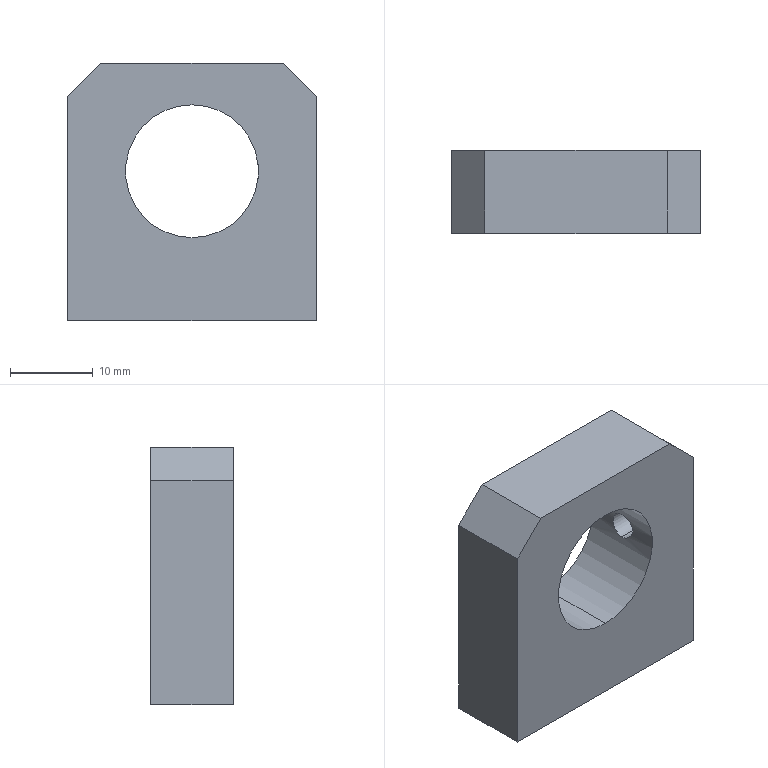Component | SolidWorks | GbgbLowerMagnetTubeFixingSeatF8-1 | 1 solid | 20 faces | box 30 x 10 x 31 mm | volume 6891 mm3 | cylinder 8 | plane 8 | cone 4 | commonest cylinder face diameters 3.3 x6 16 x2
build123d program:
from build123d import *

# Parameters (mm, degrees)
SKETCH1_W             = 30
SKETCH1_H             = 55
BOSS_EXTRUDE1_DEPTH   = 5
M4_TAPPED_HOLE2_D     = 3.3
M4_TAPPED_HOLE2_DEPTH = 10.1
M4_TAPPED_HOLE2_TIP   = 0.9914
SKETCH12_R            = 8
CUT_EXTRUDE2_DEPTH    = 12
M4_TAPPED_HOLE3_D     = 3.3
M4_TAPPED_HOLE3_DEPTH = 10.1
M4_TAPPED_HOLE3_TIP   = 0.9914
SKETCH17_W            = 30
SKETCH17_H            = 24
CUT_EXTRUDE3_DEPTH    = 10
CHAMFER1_SIZE         = 4


with BuildPart() as part:
    # Sketch1 → Boss-Extrude1 (new, symmetric)
    with BuildSketch(Plane(origin=(0, 0, 0), x_dir=(1, 0, 0), z_dir=(0, 1, 0))):
        Rectangle(SKETCH1_W, SKETCH1_H)
    extrude(amount=BOSS_EXTRUDE1_DEPTH, both=True)

    # M4 Tapped Hole2
    with Locations(Plane(origin=(2.316, -9.359, -27.5), x_dir=(1, 0, 0), z_dir=(0, 0, -1))):
        with Locations((7.684, -9.359), (-12.316, -9.359)):
            Hole(M4_TAPPED_HOLE2_D / 2, depth=M4_TAPPED_HOLE2_DEPTH)
            with Locations((0, 0, -(M4_TAPPED_HOLE2_DEPTH + M4_TAPPED_HOLE2_TIP / 2))):  # 118° drill point
                Cone(0, M4_TAPPED_HOLE2_D / 2, M4_TAPPED_HOLE2_TIP, mode=Mode.SUBTRACT)

    # Sketch12 → Cut-Extrude2 (cut)
    with BuildSketch(Plane(origin=(0, 5, 0), x_dir=(1, 0, 0), z_dir=(0, 1, 0))):
        with Locations(Location((0, 9.5, 0), (0, 0, 270))):
            Circle(SKETCH12_R)
    extrude(amount=-CUT_EXTRUDE2_DEPTH, mode=Mode.SUBTRACT)

    # M4 Tapped Hole3
    with Locations(Plane(origin=(15, 0, 0), x_dir=(0, 0, -1), z_dir=(1, 0, 0))):
        with Locations((9.5, 0)):
            Hole(M4_TAPPED_HOLE3_D / 2, depth=M4_TAPPED_HOLE3_DEPTH)
            with Locations((0, 0, -(M4_TAPPED_HOLE3_DEPTH + M4_TAPPED_HOLE3_TIP / 2))):  # 118° drill point
                Cone(0, M4_TAPPED_HOLE3_D / 2, M4_TAPPED_HOLE3_TIP, mode=Mode.SUBTRACT)

    # Sketch17 → Cut-Extrude3 (cut)
    with BuildSketch(Plane(origin=(0, 5, 0), x_dir=(1, 0, 0), z_dir=(0, 1, 0))):
        with Locations((0, -15.5)):
            Rectangle(SKETCH17_W, SKETCH17_H)
    extrude(amount=-CUT_EXTRUDE3_DEPTH, mode=Mode.SUBTRACT)

    # Chamfer1
    chamfer1_edges = [part.edges().sort_by_distance(p)[0] for p in [
        (-15, 0, 3.5),
        (15, 0, 3.5),
    ]]
    chamfer(chamfer1_edges, length=CHAMFER1_SIZE)


solid = part.part

# Placed as in the assembly
solid = solid.moved(Location((80.446, 414.94, 417.732), (0, 0, 0)))
STEP:
#1=COLOUR_RGB('',0.7922,0.8196,0.9333);
#2=FILL_AREA_STYLE_COLOUR('',#1);
#3=FILL_AREA_STYLE('',(#2));
#4=SURFACE_STYLE_FILL_AREA(#3);
#5=SURFACE_SIDE_STYLE('',(#4));
#6=SURFACE_STYLE_USAGE(.BOTH.,#5);
#7=PRESENTATION_STYLE_ASSIGNMENT((#6));
#8=CARTESIAN_POINT('',(3.475,16.336,16.137));
#9=VERTEX_POINT('',#8);
#10=CARTESIAN_POINT('',(3.475,16.336,16.007));
#11=VERTEX_POINT('',#10);
#12=CARTESIAN_POINT('',(3.475,16.336,16.137));
#13=CARTESIAN_POINT('',(3.475,16.328,16.137));
#14=CARTESIAN_POINT('',(3.476,16.319,16.135));
#15=CARTESIAN_POINT('',(3.477,16.307,16.13));
#16=CARTESIAN_POINT('',(3.477,16.304,16.128));
#17=CARTESIAN_POINT('',(3.478,16.297,16.124));
#18=CARTESIAN_POINT('',(3.478,16.293,16.121));
#19=CARTESIAN_POINT('',(3.479,16.287,16.115));
#20=CARTESIAN_POINT('',(3.48,16.285,16.112));
#21=CARTESIAN_POINT('',(3.48,16.28,16.105));
#22=CARTESIAN_POINT('',(3.481,16.278,16.101));
#23=CARTESIAN_POINT('',(3.482,16.273,16.089));
#24=CARTESIAN_POINT('',(3.482,16.271,16.081));
#25=CARTESIAN_POINT('',(3.482,16.271,16.068));
#26=CARTESIAN_POINT('',(3.482,16.272,16.064));
#27=CARTESIAN_POINT('',(3.482,16.273,16.055));
#28=CARTESIAN_POINT('',(3.481,16.275,16.051));
#29=CARTESIAN_POINT('',(3.481,16.278,16.043));
#30=CARTESIAN_POINT('',(3.48,16.28,16.04));
#31=CARTESIAN_POINT('',(3.48,16.285,16.033));
#32=CARTESIAN_POINT('',(3.479,16.287,16.029));
#33=CARTESIAN_POINT('',(3.478,16.296,16.02));
#34=CARTESIAN_POINT('',(3.477,16.303,16.015));
#35=CARTESIAN_POINT('',(3.476,16.315,16.011));
#36=CARTESIAN_POINT('',(3.476,16.319,16.009));
#37=CARTESIAN_POINT('',(3.475,16.328,16.008));
#38=CARTESIAN_POINT('',(3.475,16.332,16.007));
#39=CARTESIAN_POINT('',(3.475,16.336,16.007));
#40=B_SPLINE_CURVE_WITH_KNOTS('',3,(#12,#13,#14,#15,#16,#17,#18,#19,#20,#21,#22,#23,#24,#25,#26,#27,#28,#29,#30,#31,#32,#33,#34,#35,#36,#37,#38,#39),.UNSPECIFIED.,.F.,.F.,(4,2,2,2,2,2,2,2,2,2,2,2,2,4),(0.005173,0.005819,0.006142,0.006465,0.006789,0.007112,0.007758,0.008081,0.008405,0.008728,0.009051,0.009697,0.01002,0.01034),.UNSPECIFIED.);
#41=EDGE_CURVE('',#9,#11,#40,.T.);
#42=ORIENTED_EDGE('',*,*,#41,.F.);
#43=CARTESIAN_POINT('',(3.758,16.336,16.137));
#44=VERTEX_POINT('',#43);
#45=CARTESIAN_POINT('',(3.758,16.336,16.137));
#46=DIRECTION('',(1.,0.,-0.));
#47=VECTOR('',#46,39.37);
#48=LINE('',#45,#47);
#49=EDGE_CURVE('',#9,#44,#48,.T.);
#50=ORIENTED_EDGE('',*,*,#49,.T.);
#51=CARTESIAN_POINT('',(3.758,16.336,16.007));
#52=VERTEX_POINT('',#51);
#53=CARTESIAN_POINT('',(3.758,16.336,16.072));
#54=DIRECTION('',(1.,0.,-0.));
#55=DIRECTION('',(0.,0.,-1.));
#56=AXIS2_PLACEMENT_3D('',#53,#54,#55);
#57=CIRCLE('',#56,0.06496);
#58=EDGE_CURVE('',#44,#52,#57,.T.);
#59=ORIENTED_EDGE('',*,*,#58,.T.);
#60=CARTESIAN_POINT('',(3.758,16.336,16.007));
#61=DIRECTION('',(1.,0.,-0.));
#62=VECTOR('',#61,39.37);
#63=LINE('',#60,#62);
#64=EDGE_CURVE('',#11,#52,#63,.T.);
#65=ORIENTED_EDGE('',*,*,#64,.F.);
#66=EDGE_LOOP('',(#42,#50,#59,#65));
#67=FACE_OUTER_BOUND('',#66,.T.);
#68=CARTESIAN_POINT('',(3.758,16.336,16.072));
#69=DIRECTION('',(1.,0.,-0.));
#70=DIRECTION('',(0.,0.,-1.));
#71=AXIS2_PLACEMENT_3D('',#68,#69,#70);
#72=CYLINDRICAL_SURFACE('',#71,0.06496);
#73=ADVANCED_FACE('',(#67),#72,.F.);
#74=CARTESIAN_POINT('',(3.167,16.139,15.757));
#75=VERTEX_POINT('',#74);
#76=CARTESIAN_POINT('',(3.167,16.139,16.387));
#77=VERTEX_POINT('',#76);
#78=CARTESIAN_POINT('',(3.167,16.139,16.072));
#79=DIRECTION('',(0.,1.,0.));
#80=DIRECTION('',(0.,0.,1.));
#81=AXIS2_PLACEMENT_3D('',#78,#79,#80);
#82=CIRCLE('',#81,0.315);
#83=EDGE_CURVE('',#75,#77,#82,.T.);
#84=ORIENTED_EDGE('',*,*,#83,.F.);
#85=CARTESIAN_POINT('',(3.167,16.533,15.757));
#86=VERTEX_POINT('',#85);
#87=CARTESIAN_POINT('',(3.167,16.061,15.757));
#88=DIRECTION('',(0.,1.,0.));
#89=VECTOR('',#88,39.37);
#90=LINE('',#87,#89);
#91=EDGE_CURVE('',#75,#86,#90,.T.);
#92=ORIENTED_EDGE('',*,*,#91,.T.);
#93=CARTESIAN_POINT('',(3.167,16.533,16.387));
#94=VERTEX_POINT('',#93);
#95=CARTESIAN_POINT('',(3.167,16.533,16.072));
#96=DIRECTION('',(0.,1.,0.));
#97=DIRECTION('',(0.,0.,1.));
#98=AXIS2_PLACEMENT_3D('',#95,#96,#97);
#99=CIRCLE('',#98,0.315);
#100=EDGE_CURVE('',#86,#94,#99,.T.);
#101=ORIENTED_EDGE('',*,*,#100,.T.);
#102=CARTESIAN_POINT('',(3.167,16.061,16.387));
#103=DIRECTION('',(0.,1.,0.));
#104=VECTOR('',#103,39.37);
#105=LINE('',#102,#104);
#106=EDGE_CURVE('',#77,#94,#105,.T.);
#107=ORIENTED_EDGE('',*,*,#106,.F.);
#108=EDGE_LOOP('',(#84,#92,#101,#107));
#109=FACE_OUTER_BOUND('',#108,.T.);
#110=CARTESIAN_POINT('',(3.167,16.061,16.072));
#111=DIRECTION('',(0.,1.,0.));
#112=DIRECTION('',(0.,0.,1.));
#113=AXIS2_PLACEMENT_3D('',#110,#111,#112);
#114=CYLINDRICAL_SURFACE('',#113,0.315);
#115=ADVANCED_FACE('',(#109),#114,.F.);
#116=CARTESIAN_POINT('',(3.626,16.336,15.761));
#117=VERTEX_POINT('',#116);
#118=CARTESIAN_POINT('',(3.496,16.336,15.761));
#119=VERTEX_POINT('',#118);
#120=CARTESIAN_POINT('',(3.561,16.336,15.761));
#121=DIRECTION('',(0.,0.,-1.));
#122=DIRECTION('',(-1.,0.,0.));
#123=AXIS2_PLACEMENT_3D('',#120,#121,#122);
#124=CIRCLE('',#123,0.06496);
#125=EDGE_CURVE('',#117,#119,#124,.T.);
#126=ORIENTED_EDGE('',*,*,#125,.F.);
#127=CARTESIAN_POINT('',(3.626,16.336,15.363));
#128=VERTEX_POINT('',#127);
#129=CARTESIAN_POINT('',(3.626,16.336,15.363));
#130=DIRECTION('',(0.,0.,-1.));
#131=VECTOR('',#130,39.37);
#132=LINE('',#129,#131);
#133=EDGE_CURVE('',#117,#128,#132,.T.);
#134=ORIENTED_EDGE('',*,*,#133,.T.);
#135=CARTESIAN_POINT('',(3.496,16.336,15.363));
#136=VERTEX_POINT('',#135);
#137=CARTESIAN_POINT('',(3.561,16.336,15.363));
#138=DIRECTION('',(0.,0.,-1.));
#139=DIRECTION('',(-1.,0.,0.));
#140=AXIS2_PLACEMENT_3D('',#137,#138,#139);
#141=CIRCLE('',#140,0.06496);
#142=EDGE_CURVE('',#128,#136,#141,.T.);
#143=ORIENTED_EDGE('',*,*,#142,.T.);
#144=CARTESIAN_POINT('',(3.496,16.336,15.363));
#145=DIRECTION('',(0.,0.,-1.));
#146=VECTOR('',#145,39.37);
#147=LINE('',#144,#146);
#148=EDGE_CURVE('',#119,#136,#147,.T.);
#149=ORIENTED_EDGE('',*,*,#148,.F.);
#150=EDGE_LOOP('',(#126,#134,#143,#149));
#151=FACE_OUTER_BOUND('',#150,.T.);
#152=CARTESIAN_POINT('',(3.561,16.336,15.363));
#153=DIRECTION('',(0.,0.,-1.));
#154=DIRECTION('',(-1.,0.,0.));
#155=AXIS2_PLACEMENT_3D('',#152,#153,#154);
#156=CYLINDRICAL_SURFACE('',#155,0.06496);
#157=ADVANCED_FACE('',(#151),#156,.F.);
#158=CARTESIAN_POINT('',(3.561,16.336,15.8));
#159=VERTEX_POINT('',#158);
#160=CARTESIAN_POINT('',(3.496,16.336,15.761));
#161=DIRECTION('',(-0.8572,0.,-0.515));
#162=VECTOR('',#161,39.37);
#163=LINE('',#160,#162);
#164=EDGE_CURVE('',#159,#119,#163,.T.);
#165=ORIENTED_EDGE('',*,*,#164,.F.);
#166=CARTESIAN_POINT('',(3.626,16.336,15.761));
#167=DIRECTION('',(0.8572,0.,-0.515));
#168=VECTOR('',#167,39.37);
#169=LINE('',#166,#168);
#170=EDGE_CURVE('',#159,#117,#169,.T.);
#171=ORIENTED_EDGE('',*,*,#170,.T.);
#172=ORIENTED_EDGE('',*,*,#125,.T.);
#173=EDGE_LOOP('',(#165,#171,#172));
#174=FACE_OUTER_BOUND('',#173,.T.);
#175=CARTESIAN_POINT('',(3.561,16.336,15.761));
#176=DIRECTION('',(0.,0.,-1.));
#177=DIRECTION('',(-1.,0.,0.));
#178=AXIS2_PLACEMENT_3D('',#175,#176,#177);
#179=CONICAL_SURFACE('',#178,0.06496,1.03);
#180=ADVANCED_FACE('',(#174),#179,.F.);
#181=CARTESIAN_POINT('',(2.838,16.336,15.761));
#182=VERTEX_POINT('',#181);
#183=CARTESIAN_POINT('',(2.709,16.336,15.761));
#184=VERTEX_POINT('',#183);
#185=CARTESIAN_POINT('',(2.773,16.336,15.761));
#186=DIRECTION('',(0.,0.,-1.));
#187=DIRECTION('',(-1.,0.,0.));
#188=AXIS2_PLACEMENT_3D('',#185,#186,#187);
#189=CIRCLE('',#188,0.06496);
#190=EDGE_CURVE('',#182,#184,#189,.T.);
#191=ORIENTED_EDGE('',*,*,#190,.F.);
#192=CARTESIAN_POINT('',(2.838,16.336,15.363));
#193=VERTEX_POINT('',#192);
#194=CARTESIAN_POINT('',(2.838,16.336,15.363));
#195=DIRECTION('',(0.,0.,-1.));
#196=VECTOR('',#195,39.37);
#197=LINE('',#194,#196);
#198=EDGE_CURVE('',#182,#193,#197,.T.);
#199=ORIENTED_EDGE('',*,*,#198,.T.);
#200=CARTESIAN_POINT('',(2.709,16.336,15.363));
#201=VERTEX_POINT('',#200);
#202=CARTESIAN_POINT('',(2.773,16.336,15.363));
#203=DIRECTION('',(0.,0.,-1.));
#204=DIRECTION('',(-1.,0.,0.));
#205=AXIS2_PLACEMENT_3D('',#202,#203,#204);
#206=CIRCLE('',#205,0.06496);
#207=EDGE_CURVE('',#193,#201,#206,.T.);
#208=ORIENTED_EDGE('',*,*,#207,.T.);
#209=CARTESIAN_POINT('',(2.709,16.336,15.363));
#210=DIRECTION('',(0.,0.,-1.));
#211=VECTOR('',#210,39.37);
#212=LINE('',#209,#211);
#213=EDGE_CURVE('',#184,#201,#212,.T.);
#214=ORIENTED_EDGE('',*,*,#213,.F.);
#215=EDGE_LOOP('',(#191,#199,#208,#214));
#216=FACE_OUTER_BOUND('',#215,.T.);
#217=CARTESIAN_POINT('',(2.773,16.336,15.363));
#218=DIRECTION('',(0.,0.,-1.));
#219=DIRECTION('',(-1.,0.,0.));
#220=AXIS2_PLACEMENT_3D('',#217,#218,#219);
#221=CYLINDRICAL_SURFACE('',#220,0.06496);
#222=ADVANCED_FACE('',(#216),#221,.F.);
#223=CARTESIAN_POINT('',(2.773,16.336,15.8));
#224=VERTEX_POINT('',#223);
#225=CARTESIAN_POINT('',(2.709,16.336,15.761));
#226=DIRECTION('',(-0.8572,0.,-0.515));
#227=VECTOR('',#226,39.37);
#228=LINE('',#225,#227);
#229=EDGE_CURVE('',#224,#184,#228,.T.);
#230=ORIENTED_EDGE('',*,*,#229,.F.);
#231=CARTESIAN_POINT('',(2.838,16.336,15.761));
#232=DIRECTION('',(0.8572,0.,-0.515));
#233=VECTOR('',#232,39.37);
#234=LINE('',#231,#233);
#235=EDGE_CURVE('',#224,#182,#234,.T.);
#236=ORIENTED_EDGE('',*,*,#235,.T.);
#237=ORIENTED_EDGE('',*,*,#190,.T.);
#238=EDGE_LOOP('',(#230,#236,#237));
#239=FACE_OUTER_BOUND('',#238,.T.);
#240=CARTESIAN_POINT('',(2.773,16.336,15.761));
#241=DIRECTION('',(0.,0.,-1.));
#242=DIRECTION('',(-1.,0.,0.));
#243=AXIS2_PLACEMENT_3D('',#240,#241,#242);
#244=CONICAL_SURFACE('',#243,0.06496,1.03);
#245=ADVANCED_FACE('',(#239),#244,.F.);
#246=CARTESIAN_POINT('',(3.758,16.336,16.072));
#247=DIRECTION('',(1.,0.,-0.));
#248=DIRECTION('',(0.,0.,-1.));
#249=AXIS2_PLACEMENT_3D('',#246,#247,#248);
#250=CIRCLE('',#249,0.06496);
#251=EDGE_CURVE('',#52,#44,#250,.T.);
#252=ORIENTED_EDGE('',*,*,#251,.F.);
#253=ORIENTED_EDGE('',*,*,#58,.F.);
#254=EDGE_LOOP('',(#252,#253));
#255=FACE_BOUND('',#254,.T.);
#256=CARTESIAN_POINT('',(3.758,16.533,16.426));
#257=VERTEX_POINT('',#256);
#258=CARTESIAN_POINT('',(3.758,16.533,15.363));
#259=VERTEX_POINT('',#258);
#260=CARTESIAN_POINT('',(3.758,16.533,15.363));
#261=DIRECTION('',(-0.,0.,-1.));
#262=VECTOR('',#261,39.37);
#263=LINE('',#260,#262);
#264=EDGE_CURVE('',#257,#259,#263,.T.);
#265=ORIENTED_EDGE('',*,*,#264,.F.);
#266=CARTESIAN_POINT('',(3.758,16.139,16.426));
#267=VERTEX_POINT('',#266);
#268=CARTESIAN_POINT('',(3.758,16.533,16.426));
#269=DIRECTION('',(0.,-1.,0.));
#270=VECTOR('',#269,39.37);
#271=LINE('',#268,#270);
#272=EDGE_CURVE('',#257,#267,#271,.T.);
#273=ORIENTED_EDGE('',*,*,#272,.T.);
#274=CARTESIAN_POINT('',(3.758,16.139,15.363));
#275=VERTEX_POINT('',#274);
#276=CARTESIAN_POINT('',(3.758,16.139,15.363));
#277=DIRECTION('',(-0.,0.,-1.));
#278=VECTOR('',#277,39.37);
#279=LINE('',#276,#278);
#280=EDGE_CURVE('',#267,#275,#279,.T.);
#281=ORIENTED_EDGE('',*,*,#280,.T.);
#282=CARTESIAN_POINT('',(3.758,16.533,15.363));
#283=DIRECTION('',(0.,-1.,0.));
#284=VECTOR('',#283,39.37);
#285=LINE('',#282,#284);
#286=EDGE_CURVE('',#259,#275,#285,.T.);
#287=ORIENTED_EDGE('',*,*,#286,.F.);
#288=EDGE_LOOP('',(#265,#273,#281,#287));
#289=FACE_OUTER_BOUND('',#288,.T.);
#290=CARTESIAN_POINT('',(3.758,16.533,15.363));
#291=DIRECTION('',(-1.,0.,0.));
#292=DIRECTION('',(0.,0.,1.));
#293=AXIS2_PLACEMENT_3D('',#290,#291,#292);
#294=PLANE('',#293);
#295=ADVANCED_FACE('',(#255,#289),#294,.F.);
#296=CARTESIAN_POINT('',(3.561,16.336,15.363));
#297=DIRECTION('',(0.,0.,-1.));
#298=DIRECTION('',(-1.,0.,0.));
#299=AXIS2_PLACEMENT_3D('',#296,#297,#298);
#300=CIRCLE('',#299,0.06496);
#301=EDGE_CURVE('',#136,#128,#300,.T.);
#302=ORIENTED_EDGE('',*,*,#301,.F.);
#303=ORIENTED_EDGE('',*,*,#142,.F.);
#304=EDGE_LOOP('',(#302,#303));
#305=FACE_BOUND('',#304,.T.);
#306=CARTESIAN_POINT('',(2.773,16.336,15.363));
#307=DIRECTION('',(0.,0.,-1.));
#308=DIRECTION('',(-1.,0.,0.));
#309=AXIS2_PLACEMENT_3D('',#306,#307,#308);
#310=CIRCLE('',#309,0.06496);
#311=EDGE_CURVE('',#201,#193,#310,.T.);
#312=ORIENTED_EDGE('',*,*,#311,.F.);
#313=ORIENTED_EDGE('',*,*,#207,.F.);
#314=EDGE_LOOP('',(#312,#313));
#315=FACE_BOUND('',#314,.T.);
#316=CARTESIAN_POINT('',(2.577,16.139,15.363));
#317=VERTEX_POINT('',#316);
#318=CARTESIAN_POINT('',(2.577,16.139,15.363));
#319=DIRECTION('',(-1.,0.,0.));
#320=VECTOR('',#319,39.37);
#321=LINE('',#318,#320);
#322=EDGE_CURVE('',#275,#317,#321,.T.);
#323=ORIENTED_EDGE('',*,*,#322,.T.);
#324=CARTESIAN_POINT('',(2.577,16.533,15.363));
#325=VERTEX_POINT('',#324);
#326=CARTESIAN_POINT('',(2.577,16.533,15.363));
#327=DIRECTION('',(0.,-1.,0.));
#328=VECTOR('',#327,39.37);
#329=LINE('',#326,#328);
#330=EDGE_CURVE('',#325,#317,#329,.T.);
#331=ORIENTED_EDGE('',*,*,#330,.F.);
#332=CARTESIAN_POINT('',(2.577,16.533,15.363));
#333=DIRECTION('',(-1.,0.,0.));
#334=VECTOR('',#333,39.37);
#335=LINE('',#332,#334);
#336=EDGE_CURVE('',#259,#325,#335,.T.);
#337=ORIENTED_EDGE('',*,*,#336,.F.);
#338=ORIENTED_EDGE('',*,*,#286,.T.);
#339=EDGE_LOOP('',(#323,#331,#337,#338));
#340=FACE_OUTER_BOUND('',#339,.T.);
#341=CARTESIAN_POINT('',(2.577,16.533,15.363));
#342=DIRECTION('',(0.,0.,1.));
#343=DIRECTION('',(1.,0.,0.));
#344=AXIS2_PLACEMENT_3D('',#341,#342,#343);
#345=PLANE('',#344);
#346=ADVANCED_FACE('',(#305,#315,#340),#345,.F.);
#347=CARTESIAN_POINT('',(2.577,16.139,16.426));
#348=VERTEX_POINT('',#347);
#349=CARTESIAN_POINT('',(2.577,16.139,15.363));
#350=DIRECTION('',(0.,0.,1.));
#351=VECTOR('',#350,39.37);
#352=LINE('',#349,#351);
#353=EDGE_CURVE('',#317,#348,#352,.T.);
#354=ORIENTED_EDGE('',*,*,#353,.T.);
#355=CARTESIAN_POINT('',(2.577,16.533,16.426));
#356=VERTEX_POINT('',#355);
#357=CARTESIAN_POINT('',(2.577,16.533,16.426));
#358=DIRECTION('',(0.,1.,0.));
#359=VECTOR('',#358,39.37);
#360=LINE('',#357,#359);
#361=EDGE_CURVE('',#348,#356,#360,.T.);
#362=ORIENTED_EDGE('',*,*,#361,.T.);
#363=CARTESIAN_POINT('',(2.577,16.533,15.363));
#364=DIRECTION('',(0.,0.,1.));
#365=VECTOR('',#364,39.37);
#366=LINE('',#363,#365);
#367=EDGE_CURVE('',#325,#356,#366,.T.);
#368=ORIENTED_EDGE('',*,*,#367,.F.);
#369=ORIENTED_EDGE('',*,*,#330,.T.);
#370=EDGE_LOOP('',(#354,#362,#368,#369));
#371=FACE_OUTER_BOUND('',#370,.T.);
#372=CARTESIAN_POINT('',(2.577,16.533,15.363));
#373=DIRECTION('',(1.,0.,-0.));
#374=DIRECTION('',(-0.,0.,-1.));
#375=AXIS2_PLACEMENT_3D('',#372,#373,#374);
#376=PLANE('',#375);
#377=ADVANCED_FACE('',(#371),#376,.F.);
#378=ORIENTED_EDGE('',*,*,#367,.T.);
#379=CARTESIAN_POINT('',(2.734,16.533,16.584));
#380=VERTEX_POINT('',#379);
#381=CARTESIAN_POINT('',(2.882,16.533,16.732));
#382=DIRECTION('',(0.7071,0.,0.7071));
#383=VECTOR('',#382,39.37);
#384=LINE('',#381,#383);
#385=EDGE_CURVE('',#356,#380,#384,.T.);
#386=ORIENTED_EDGE('',*,*,#385,.T.);
#387=CARTESIAN_POINT('',(3.6,16.533,16.584));
#388=VERTEX_POINT('',#387);
#389=CARTESIAN_POINT('',(2.577,16.533,16.584));
#390=DIRECTION('',(-1.,0.,0.));
#391=VECTOR('',#390,39.37);
#392=LINE('',#389,#391);
#393=EDGE_CURVE('',#388,#380,#392,.T.);
#394=ORIENTED_EDGE('',*,*,#393,.F.);
#395=CARTESIAN_POINT('',(3.453,16.533,16.732));
#396=DIRECTION('',(0.7071,0.,-0.7071));
#397=VECTOR('',#396,39.37);
#398=LINE('',#395,#397);
#399=EDGE_CURVE('',#388,#257,#398,.T.);
#400=ORIENTED_EDGE('',*,*,#399,.T.);
#401=ORIENTED_EDGE('',*,*,#264,.T.);
#402=ORIENTED_EDGE('',*,*,#336,.T.);
#403=EDGE_LOOP('',(#378,#386,#394,#400,#401,#402));
#404=FACE_OUTER_BOUND('',#403,.T.);
#405=CARTESIAN_POINT('',(3.167,16.533,16.072));
#406=DIRECTION('',(0.,1.,0.));
#407=DIRECTION('',(0.,0.,1.));
#408=AXIS2_PLACEMENT_3D('',#405,#406,#407);
#409=CIRCLE('',#408,0.315);
#410=EDGE_CURVE('',#94,#86,#409,.T.);
#411=ORIENTED_EDGE('',*,*,#410,.F.);
#412=ORIENTED_EDGE('',*,*,#100,.F.);
#413=EDGE_LOOP('',(#411,#412));
#414=FACE_BOUND('',#413,.T.);
#415=CARTESIAN_POINT('',(3.167,16.533,16.446));
#416=DIRECTION('',(0.,1.,0.));
#417=DIRECTION('',(0.,0.,1.));
#418=AXIS2_PLACEMENT_3D('',#415,#416,#417);
#419=PLANE('',#418);
#420=ADVANCED_FACE('',(#404,#414),#419,.T.);
#421=CARTESIAN_POINT('',(3.167,16.139,16.072));
#422=DIRECTION('',(0.,1.,0.));
#423=DIRECTION('',(0.,0.,1.));
#424=AXIS2_PLACEMENT_3D('',#421,#422,#423);
#425=CIRCLE('',#424,0.315);
#426=EDGE_CURVE('',#77,#75,#425,.T.);
#427=ORIENTED_EDGE('',*,*,#426,.T.);
#428=ORIENTED_EDGE('',*,*,#83,.T.);
#429=EDGE_LOOP('',(#427,#428));
#430=FACE_BOUND('',#429,.T.);
#431=CARTESIAN_POINT('',(3.6,16.139,16.584));
#432=VERTEX_POINT('',#431);
#433=CARTESIAN_POINT('',(2.734,16.139,16.584));
#434=VERTEX_POINT('',#433);
#435=CARTESIAN_POINT('',(2.577,16.139,16.584));
#436=DIRECTION('',(-1.,0.,0.));
#437=VECTOR('',#436,39.37);
#438=LINE('',#435,#437);
#439=EDGE_CURVE('',#432,#434,#438,.T.);
#440=ORIENTED_EDGE('',*,*,#439,.T.);
#441=CARTESIAN_POINT('',(2.577,16.139,16.426));
#442=DIRECTION('',(-0.7071,0.,-0.7071));
#443=VECTOR('',#442,39.37);
#444=LINE('',#441,#443);
#445=EDGE_CURVE('',#434,#348,#444,.T.);
#446=ORIENTED_EDGE('',*,*,#445,.T.);
#447=ORIENTED_EDGE('',*,*,#353,.F.);
#448=ORIENTED_EDGE('',*,*,#322,.F.);
#449=ORIENTED_EDGE('',*,*,#280,.F.);
#450=CARTESIAN_POINT('',(3.6,16.139,16.584));
#451=DIRECTION('',(-0.7071,0.,0.7071));
#452=VECTOR('',#451,39.37);
#453=LINE('',#450,#452);
#454=EDGE_CURVE('',#267,#432,#453,.T.);
#455=ORIENTED_EDGE('',*,*,#454,.T.);
#456=EDGE_LOOP('',(#440,#446,#447,#448,#449,#455));
#457=FACE_OUTER_BOUND('',#456,.T.);
#458=CARTESIAN_POINT('',(3.167,16.139,16.446));
#459=DIRECTION('',(0.,1.,0.));
#460=DIRECTION('',(0.,0.,1.));
#461=AXIS2_PLACEMENT_3D('',#458,#459,#460);
#462=PLANE('',#461);
#463=ADVANCED_FACE('',(#430,#457),#462,.F.);
#464=ORIENTED_EDGE('',*,*,#235,.F.);
#465=ORIENTED_EDGE('',*,*,#229,.T.);
#466=CARTESIAN_POINT('',(2.773,16.336,15.761));
#467=DIRECTION('',(0.,0.,-1.));
#468=DIRECTION('',(-1.,0.,0.));
#469=AXIS2_PLACEMENT_3D('',#466,#467,#468);
#470=CIRCLE('',#469,0.06496);
#471=EDGE_CURVE('',#184,#182,#470,.T.);
#472=ORIENTED_EDGE('',*,*,#471,.T.);
#473=EDGE_LOOP('',(#464,#465,#472));
#474=FACE_OUTER_BOUND('',#473,.T.);
#475=CARTESIAN_POINT('',(2.773,16.336,15.761));
#476=DIRECTION('',(0.,0.,-1.));
#477=DIRECTION('',(-1.,0.,0.));
#478=AXIS2_PLACEMENT_3D('',#475,#476,#477);
#479=CONICAL_SURFACE('',#478,0.06496,1.03);
#480=ADVANCED_FACE('',(#474),#479,.F.);
#481=ORIENTED_EDGE('',*,*,#198,.F.);
#482=ORIENTED_EDGE('',*,*,#471,.F.);
#483=ORIENTED_EDGE('',*,*,#213,.T.);
#484=ORIENTED_EDGE('',*,*,#311,.T.);
#485=EDGE_LOOP('',(#481,#482,#483,#484));
#486=FACE_OUTER_BOUND('',#485,.T.);
#487=CARTESIAN_POINT('',(2.773,16.336,15.363));
#488=DIRECTION('',(0.,0.,-1.));
#489=DIRECTION('',(-1.,0.,0.));
#490=AXIS2_PLACEMENT_3D('',#487,#488,#489);
#491=CYLINDRICAL_SURFACE('',#490,0.06496);
#492=ADVANCED_FACE('',(#486),#491,.F.);
#493=ORIENTED_EDGE('',*,*,#170,.F.);
#494=ORIENTED_EDGE('',*,*,#164,.T.);
#495=CARTESIAN_POINT('',(3.561,16.336,15.761));
#496=DIRECTION('',(0.,0.,-1.));
#497=DIRECTION('',(-1.,0.,0.));
#498=AXIS2_PLACEMENT_3D('',#495,#496,#497);
#499=CIRCLE('',#498,0.06496);
#500=EDGE_CURVE('',#119,#117,#499,.T.);
#501=ORIENTED_EDGE('',*,*,#500,.T.);
#502=EDGE_LOOP('',(#493,#494,#501));
#503=FACE_OUTER_BOUND('',#502,.T.);
#504=CARTESIAN_POINT('',(3.561,16.336,15.761));
#505=DIRECTION('',(0.,0.,-1.));
#506=DIRECTION('',(-1.,0.,0.));
#507=AXIS2_PLACEMENT_3D('',#504,#505,#506);
#508=CONICAL_SURFACE('',#507,0.06496,1.03);
#509=ADVANCED_FACE('',(#503),#508,.F.);
#510=ORIENTED_EDGE('',*,*,#133,.F.);
#511=ORIENTED_EDGE('',*,*,#500,.F.);
#512=ORIENTED_EDGE('',*,*,#148,.T.);
#513=ORIENTED_EDGE('',*,*,#301,.T.);
#514=EDGE_LOOP('',(#510,#511,#512,#513));
#515=FACE_OUTER_BOUND('',#514,.T.);
#516=CARTESIAN_POINT('',(3.561,16.336,15.363));
#517=DIRECTION('',(0.,0.,-1.));
#518=DIRECTION('',(-1.,0.,0.));
#519=AXIS2_PLACEMENT_3D('',#516,#517,#518);
#520=CYLINDRICAL_SURFACE('',#519,0.06496);
#521=ADVANCED_FACE('',(#515),#520,.F.);
#522=ORIENTED_EDGE('',*,*,#91,.F.);
#523=ORIENTED_EDGE('',*,*,#426,.F.);
#524=ORIENTED_EDGE('',*,*,#106,.T.);
#525=ORIENTED_EDGE('',*,*,#410,.T.);
#526=EDGE_LOOP('',(#522,#523,#524,#525));
#527=FACE_OUTER_BOUND('',#526,.T.);
#528=CARTESIAN_POINT('',(3.475,16.336,16.007));
#529=CARTESIAN_POINT('',(3.475,16.341,16.007));
#530=CARTESIAN_POINT('',(3.475,16.345,16.008));
#531=CARTESIAN_POINT('',(3.476,16.353,16.009));
#532=CARTESIAN_POINT('',(3.476,16.357,16.01));
#533=CARTESIAN_POINT('',(3.477,16.365,16.014));
#534=CARTESIAN_POINT('',(3.477,16.369,16.016));
#535=CARTESIAN_POINT('',(3.478,16.376,16.02));
#536=CARTESIAN_POINT('',(3.478,16.379,16.023));
#537=CARTESIAN_POINT('',(3.48,16.388,16.032));
#538=CARTESIAN_POINT('',(3.481,16.393,16.039));
#539=CARTESIAN_POINT('',(3.482,16.399,16.055));
#540=CARTESIAN_POINT('',(3.482,16.401,16.064));
#541=CARTESIAN_POINT('',(3.482,16.401,16.076));
#542=CARTESIAN_POINT('',(3.482,16.401,16.081));
#543=CARTESIAN_POINT('',(3.482,16.399,16.089));
#544=CARTESIAN_POINT('',(3.481,16.398,16.093));
#545=CARTESIAN_POINT('',(3.481,16.393,16.105));
#546=CARTESIAN_POINT('',(3.48,16.388,16.112));
#547=CARTESIAN_POINT('',(3.478,16.379,16.121));
#548=CARTESIAN_POINT('',(3.478,16.376,16.124));
#549=CARTESIAN_POINT('',(3.477,16.369,16.128));
#550=CARTESIAN_POINT('',(3.477,16.365,16.13));
#551=CARTESIAN_POINT('',(3.476,16.357,16.134));
#552=CARTESIAN_POINT('',(3.476,16.353,16.135));
#553=CARTESIAN_POINT('',(3.475,16.345,16.137));
#554=CARTESIAN_POINT('',(3.475,16.34,16.137));
#555=CARTESIAN_POINT('',(3.475,16.336,16.137));
#556=B_SPLINE_CURVE_WITH_KNOTS('',3,(#528,#529,#530,#531,#532,#533,#534,#535,#536,#537,#538,#539,#540,#541,#542,#543,#544,#545,#546,#547,#548,#549,#550,#551,#552,#553,#554,#555),.UNSPECIFIED.,.F.,.F.,(4,2,2,2,2,2,2,2,2,2,2,2,2,4),(0.,0.0003233,0.0006466,0.0009699,0.001293,0.00194,0.002586,0.00291,0.003233,0.003879,0.004203,0.004526,0.004849,0.005173),.UNSPECIFIED.);
#557=EDGE_CURVE('',#11,#9,#556,.T.);
#558=ORIENTED_EDGE('',*,*,#557,.T.);
#559=ORIENTED_EDGE('',*,*,#41,.T.);
#560=EDGE_LOOP('',(#558,#559));
#561=FACE_BOUND('',#560,.T.);
#562=CARTESIAN_POINT('',(3.167,16.061,16.072));
#563=DIRECTION('',(0.,1.,0.));
#564=DIRECTION('',(0.,0.,1.));
#565=AXIS2_PLACEMENT_3D('',#562,#563,#564);
#566=CYLINDRICAL_SURFACE('',#565,0.315);
#567=ADVANCED_FACE('',(#527,#561),#566,.F.);
#568=ORIENTED_EDGE('',*,*,#49,.F.);
#569=ORIENTED_EDGE('',*,*,#557,.F.);
#570=ORIENTED_EDGE('',*,*,#64,.T.);
#571=ORIENTED_EDGE('',*,*,#251,.T.);
#572=EDGE_LOOP('',(#568,#569,#570,#571));
#573=FACE_OUTER_BOUND('',#572,.T.);
#574=CARTESIAN_POINT('',(3.758,16.336,16.072));
#575=DIRECTION('',(1.,0.,-0.));
#576=DIRECTION('',(0.,0.,-1.));
#577=AXIS2_PLACEMENT_3D('',#574,#575,#576);
#578=CYLINDRICAL_SURFACE('',#577,0.06496);
#579=ADVANCED_FACE('',(#573),#578,.F.);
#580=ORIENTED_EDGE('',*,*,#393,.T.);
#581=CARTESIAN_POINT('',(2.734,16.139,16.584));
#582=DIRECTION('',(0.,-1.,0.));
#583=VECTOR('',#582,39.37);
#584=LINE('',#581,#583);
#585=EDGE_CURVE('',#380,#434,#584,.T.);
#586=ORIENTED_EDGE('',*,*,#585,.T.);
#587=ORIENTED_EDGE('',*,*,#439,.F.);
#588=CARTESIAN_POINT('',(3.6,16.139,16.584));
#589=DIRECTION('',(0.,1.,0.));
#590=VECTOR('',#589,39.37);
#591=LINE('',#588,#590);
#592=EDGE_CURVE('',#432,#388,#591,.T.);
#593=ORIENTED_EDGE('',*,*,#592,.T.);
#594=EDGE_LOOP('',(#580,#586,#587,#593));
#595=FACE_OUTER_BOUND('',#594,.T.);
#596=CARTESIAN_POINT('',(2.577,16.139,16.584));
#597=DIRECTION('',(0.,0.,-1.));
#598=DIRECTION('',(-1.,0.,0.));
#599=AXIS2_PLACEMENT_3D('',#596,#597,#598);
#600=PLANE('',#599);
#601=ADVANCED_FACE('',(#595),#600,.F.);
#602=ORIENTED_EDGE('',*,*,#445,.F.);
#603=ORIENTED_EDGE('',*,*,#585,.F.);
#604=ORIENTED_EDGE('',*,*,#385,.F.);
#605=ORIENTED_EDGE('',*,*,#361,.F.);
#606=EDGE_LOOP('',(#602,#603,#604,#605));
#607=FACE_OUTER_BOUND('',#606,.T.);
#608=CARTESIAN_POINT('',(2.577,16.533,16.426));
#609=DIRECTION('',(0.7071,0.,-0.7071));
#610=DIRECTION('',(0.,1.,0.));
#611=AXIS2_PLACEMENT_3D('',#608,#609,#610);
#612=PLANE('',#611);
#613=ADVANCED_FACE('',(#607),#612,.F.);
#614=ORIENTED_EDGE('',*,*,#454,.F.);
#615=ORIENTED_EDGE('',*,*,#272,.F.);
#616=ORIENTED_EDGE('',*,*,#399,.F.);
#617=ORIENTED_EDGE('',*,*,#592,.F.);
#618=EDGE_LOOP('',(#614,#615,#616,#617));
#619=FACE_OUTER_BOUND('',#618,.T.);
#620=CARTESIAN_POINT('',(3.6,16.139,16.584));
#621=DIRECTION('',(-0.7071,0.,-0.7071));
#622=DIRECTION('',(0.,1.,0.));
#623=AXIS2_PLACEMENT_3D('',#620,#621,#622);
#624=PLANE('',#623);
#625=ADVANCED_FACE('',(#619),#624,.F.);
#626=CLOSED_SHELL('',(#73,#115,#157,#180,#222,#245,#295,#346,#377,#420,#463,#480,#492,#509,#521,#567,#579,#601,#613,#625));
#627=MANIFOLD_SOLID_BREP('',#626);
#628=STYLED_ITEM('',(#7),#627);
#629=PRESENTATION_LAYER_ASSIGNMENT('','',(#628));
#630=(LENGTH_UNIT()NAMED_UNIT(*)SI_UNIT($,.METRE.));
#631=LENGTH_MEASURE_WITH_UNIT(LENGTH_MEASURE(0.0254),#630);
#632=DIMENSIONAL_EXPONENTS(1.,0.,0.,0.,0.,0.,0.);
#633=(CONVERSION_BASED_UNIT('',#631)LENGTH_UNIT()NAMED_UNIT(#632));
#634=UNCERTAINTY_MEASURE_WITH_UNIT(LENGTH_MEASURE(0.00001),#633,'','');
#635=(NAMED_UNIT(*)PLANE_ANGLE_UNIT()SI_UNIT($,.RADIAN.));
#636=(NAMED_UNIT(*)SI_UNIT($,.STERADIAN.)SOLID_ANGLE_UNIT());
#637=(GEOMETRIC_REPRESENTATION_CONTEXT(3)GLOBAL_UNCERTAINTY_ASSIGNED_CONTEXT((#634))GLOBAL_UNIT_ASSIGNED_CONTEXT((#633,#635,#636))REPRESENTATION_CONTEXT('',''));
#638=MECHANICAL_DESIGN_GEOMETRIC_PRESENTATION_REPRESENTATION('',(#628),#637);
#639=CARTESIAN_POINT('',(0.,0.,0.));
#640=DIRECTION('',(0.,0.,1.));
#641=DIRECTION('',(1.,0.,0.));
#642=AXIS2_PLACEMENT_3D('',#639,#640,#641);
#643=(LENGTH_UNIT()NAMED_UNIT(*)SI_UNIT($,.METRE.));
#644=LENGTH_MEASURE_WITH_UNIT(LENGTH_MEASURE(0.0254),#643);
#645=DIMENSIONAL_EXPONENTS(1.,0.,0.,0.,0.,0.,0.);
#646=(CONVERSION_BASED_UNIT('',#644)LENGTH_UNIT()NAMED_UNIT(#645));
#647=UNCERTAINTY_MEASURE_WITH_UNIT(LENGTH_MEASURE(0.00001),#646,'','');
#648=(NAMED_UNIT(*)PLANE_ANGLE_UNIT()SI_UNIT($,.RADIAN.));
#649=(NAMED_UNIT(*)SI_UNIT($,.STERADIAN.)SOLID_ANGLE_UNIT());
#650=(GEOMETRIC_REPRESENTATION_CONTEXT(3)GLOBAL_UNCERTAINTY_ASSIGNED_CONTEXT((#647))GLOBAL_UNIT_ASSIGNED_CONTEXT((#646,#648,#649))REPRESENTATION_CONTEXT('',''));
#651=ADVANCED_BREP_SHAPE_REPRESENTATION('',(#627,#642),#650);